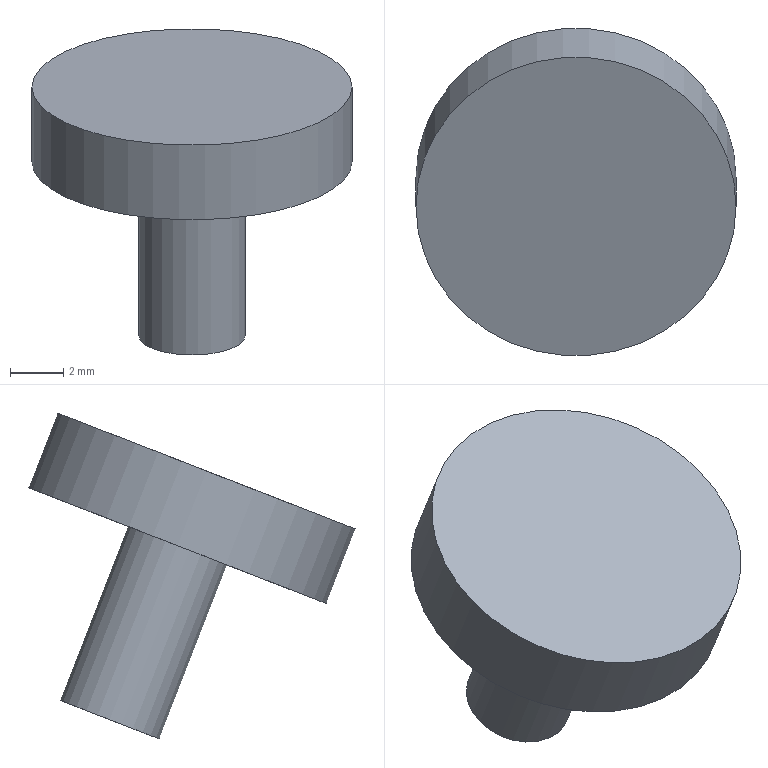Component | NX | 23G__27 | 1 solid | 5 faces | box 12 x 12.27 x 12.22 mm | volume 427 mm3 | plane 3 | cylinder 2 | commonest cylinder face diameters 4 x1 12 x1
STEP:
#1=CARTESIAN_POINT('',(0.,0.,0.));
#2=DIRECTION('',(0.,0.,1.));
#3=DIRECTION('',(1.,0.,0.));
#4=AXIS2_PLACEMENT_3D('',#1,#2,#3);
#5=CARTESIAN_POINT('',(19.022,57.969,101.64));
#6=VERTEX_POINT('',#5);
#7=CARTESIAN_POINT('',(17.022,57.969,101.64));
#8=DIRECTION('',(0.,-0.3629,0.9318));
#9=DIRECTION('',(1.,0.,0.));
#10=AXIS2_PLACEMENT_3D('',#7,#8,#9);
#11=CIRCLE('',#10,2.);
#12=CARTESIAN_POINT('',(17.022,57.969,101.64));
#13=DIRECTION('',(0.,-0.3629,0.9318));
#14=DIRECTION('',(1.,0.,0.));
#15=AXIS2_PLACEMENT_3D('',#12,#13,#14);
#16=PLANE('',#15);
#17=CARTESIAN_POINT('',(0.,0.));
#18=DIRECTION('',(1.,0.));
#19=AXIS2_PLACEMENT_2D('',#17,#18);
#20=CIRCLE('',#19,2.);
#21=(GEOMETRIC_REPRESENTATION_CONTEXT(2)PARAMETRIC_REPRESENTATION_CONTEXT()REPRESENTATION_CONTEXT('',''));
#22=DEFINITIONAL_REPRESENTATION('',(#20),#21);
#23=PCURVE('',#16,#22);
#24=CARTESIAN_POINT('',(17.022,57.969,101.64));
#25=DIRECTION('',(0.,-0.3629,0.9318));
#26=DIRECTION('',(1.,0.,0.));
#27=AXIS2_PLACEMENT_3D('',#24,#25,#26);
#28=CYLINDRICAL_SURFACE('',#27,2.);
#29=CARTESIAN_POINT('',(0.,0.));
#30=DIRECTION('',(1.,0.));
#31=VECTOR('',#30,1.);
#32=LINE('',#29,#31);
#33=(GEOMETRIC_REPRESENTATION_CONTEXT(2)PARAMETRIC_REPRESENTATION_CONTEXT()REPRESENTATION_CONTEXT('',''));
#34=DEFINITIONAL_REPRESENTATION('',(#32),#33);
#35=PCURVE('',#28,#34);
#36=SURFACE_CURVE('',#11,(#23,#35),.PCURVE_S1.);
#37=EDGE_CURVE('',#6,#6,#36,.T.);
#38=ORIENTED_EDGE('',*,*,#37,.F.);
#39=EDGE_LOOP('',(#38));
#40=FACE_BOUND('',#39,.T.);
#41=ADVANCED_FACE('',(#40),#16,.F.);
#42=CARTESIAN_POINT('',(19.022,55.429,108.162));
#43=VERTEX_POINT('',#42);
#44=CARTESIAN_POINT('',(17.022,55.429,108.162));
#45=DIRECTION('',(0.,-0.3629,0.9318));
#46=DIRECTION('',(1.,0.,0.));
#47=AXIS2_PLACEMENT_3D('',#44,#45,#46);
#48=CIRCLE('',#47,2.);
#49=CARTESIAN_POINT('',(0.,7.));
#50=DIRECTION('',(1.,0.));
#51=VECTOR('',#50,1.);
#52=LINE('',#49,#51);
#53=(GEOMETRIC_REPRESENTATION_CONTEXT(2)PARAMETRIC_REPRESENTATION_CONTEXT()REPRESENTATION_CONTEXT('',''));
#54=DEFINITIONAL_REPRESENTATION('',(#52),#53);
#55=PCURVE('',#28,#54);
#56=CARTESIAN_POINT('',(17.022,57.292,108.888));
#57=DIRECTION('',(0.,-0.3629,0.9318));
#58=DIRECTION('',(1.,0.,0.));
#59=AXIS2_PLACEMENT_3D('',#56,#57,#58);
#60=PLANE('',#59);
#61=CARTESIAN_POINT('',(0.,-2.));
#62=DIRECTION('',(1.,0.));
#63=AXIS2_PLACEMENT_2D('',#61,#62);
#64=CIRCLE('',#63,2.);
#65=(GEOMETRIC_REPRESENTATION_CONTEXT(2)PARAMETRIC_REPRESENTATION_CONTEXT()REPRESENTATION_CONTEXT('',''));
#66=DEFINITIONAL_REPRESENTATION('',(#64),#65);
#67=PCURVE('',#60,#66);
#68=SURFACE_CURVE('',#48,(#55,#67),.PCURVE_S1.);
#69=EDGE_CURVE('',#43,#43,#68,.T.);
#70=ORIENTED_EDGE('',*,*,#69,.F.);
#71=CARTESIAN_POINT('',(19.022,57.969,101.64));
#72=CARTESIAN_POINT('',(19.022,55.429,108.162));
#73=B_SPLINE_CURVE_WITH_KNOTS('',1,(#71,#72),.UNSPECIFIED.,.F.,.F.,(2,2),(0.,7.),.PIECEWISE_BEZIER_KNOTS.);
#74=CARTESIAN_POINT('',(0.,0.));
#75=DIRECTION('',(0.,1.));
#76=VECTOR('',#75,1.);
#77=LINE('',#74,#76);
#78=(GEOMETRIC_REPRESENTATION_CONTEXT(2)PARAMETRIC_REPRESENTATION_CONTEXT()REPRESENTATION_CONTEXT('',''));
#79=DEFINITIONAL_REPRESENTATION('',(#77),#78);
#80=PCURVE('',#28,#79);
#81=CARTESIAN_POINT('',(6.283,0.));
#82=DIRECTION('',(0.,1.));
#83=VECTOR('',#82,1.);
#84=LINE('',#81,#83);
#85=(GEOMETRIC_REPRESENTATION_CONTEXT(2)PARAMETRIC_REPRESENTATION_CONTEXT()REPRESENTATION_CONTEXT('',''));
#86=DEFINITIONAL_REPRESENTATION('',(#84),#85);
#87=PCURVE('',#28,#86);
#88=SEAM_CURVE('',#73,(#80,#87),.PCURVE_S1.);
#89=EDGE_CURVE('',#6,#43,#88,.T.);
#90=ORIENTED_EDGE('',*,*,#89,.F.);
#91=ORIENTED_EDGE('',*,*,#37,.T.);
#92=ORIENTED_EDGE('',*,*,#89,.T.);
#93=EDGE_LOOP('',(#70,#90,#91,#92));
#94=FACE_BOUND('',#93,.T.);
#95=ADVANCED_FACE('',(#94),#28,.T.);
#96=CARTESIAN_POINT('',(23.022,55.429,108.162));
#97=VERTEX_POINT('',#96);
#98=CARTESIAN_POINT('',(17.022,55.429,108.162));
#99=DIRECTION('',(0.,-0.3629,0.9318));
#100=DIRECTION('',(1.,0.,0.));
#101=AXIS2_PLACEMENT_3D('',#98,#99,#100);
#102=CIRCLE('',#101,6.);
#103=CARTESIAN_POINT('',(0.,-2.));
#104=DIRECTION('',(1.,0.));
#105=AXIS2_PLACEMENT_2D('',#103,#104);
#106=CIRCLE('',#105,6.);
#107=(GEOMETRIC_REPRESENTATION_CONTEXT(2)PARAMETRIC_REPRESENTATION_CONTEXT()REPRESENTATION_CONTEXT('',''));
#108=DEFINITIONAL_REPRESENTATION('',(#106),#107);
#109=PCURVE('',#60,#108);
#110=CARTESIAN_POINT('',(17.022,57.969,101.64));
#111=DIRECTION('',(0.,-0.3629,0.9318));
#112=DIRECTION('',(1.,0.,0.));
#113=AXIS2_PLACEMENT_3D('',#110,#111,#112);
#114=CYLINDRICAL_SURFACE('',#113,6.);
#115=CARTESIAN_POINT('',(0.,7.));
#116=DIRECTION('',(1.,0.));
#117=VECTOR('',#116,1.);
#118=LINE('',#115,#117);
#119=(GEOMETRIC_REPRESENTATION_CONTEXT(2)PARAMETRIC_REPRESENTATION_CONTEXT()REPRESENTATION_CONTEXT('',''));
#120=DEFINITIONAL_REPRESENTATION('',(#118),#119);
#121=PCURVE('',#114,#120);
#122=SURFACE_CURVE('',#102,(#109,#121),.PCURVE_S1.);
#123=EDGE_CURVE('',#97,#97,#122,.T.);
#124=ORIENTED_EDGE('',*,*,#123,.F.);
#125=EDGE_LOOP('',(#124));
#126=FACE_BOUND('',#125,.T.);
#127=ORIENTED_EDGE('',*,*,#69,.T.);
#128=EDGE_LOOP('',(#127));
#129=FACE_BOUND('',#128,.T.);
#130=ADVANCED_FACE('',(#126,#129),#60,.F.);
#131=CARTESIAN_POINT('',(23.022,54.34,110.958));
#132=VERTEX_POINT('',#131);
#133=CARTESIAN_POINT('',(17.022,54.34,110.958));
#134=DIRECTION('',(0.,-0.3629,0.9318));
#135=DIRECTION('',(1.,0.,0.));
#136=AXIS2_PLACEMENT_3D('',#133,#134,#135);
#137=CIRCLE('',#136,6.);
#138=CARTESIAN_POINT('',(0.,10.));
#139=DIRECTION('',(1.,0.));
#140=VECTOR('',#139,1.);
#141=LINE('',#138,#140);
#142=(GEOMETRIC_REPRESENTATION_CONTEXT(2)PARAMETRIC_REPRESENTATION_CONTEXT()REPRESENTATION_CONTEXT('',''));
#143=DEFINITIONAL_REPRESENTATION('',(#141),#142);
#144=PCURVE('',#114,#143);
#145=CARTESIAN_POINT('',(17.022,59.931,113.135));
#146=DIRECTION('',(0.,0.3629,-0.9318));
#147=DIRECTION('',(-1.,0.,0.));
#148=AXIS2_PLACEMENT_3D('',#145,#146,#147);
#149=PLANE('',#148);
#150=CARTESIAN_POINT('',(-6.,-6.));
#151=CARTESIAN_POINT('',(-6.,4.392));
#152=CARTESIAN_POINT('',(3.,-0.8038));
#153=CARTESIAN_POINT('',(12.,-6.));
#154=CARTESIAN_POINT('',(3.,-11.196));
#155=CARTESIAN_POINT('',(-6.,-16.392));
#156=CARTESIAN_POINT('',(-6.,-6.));
#157=(BOUNDED_CURVE()B_SPLINE_CURVE(2,(#150,#151,#152,#153,#154,#155,#156),.UNSPECIFIED.,.T.,.F.)B_SPLINE_CURVE_WITH_KNOTS((1,2,2,2,2,1),(-2.094,0.,2.094,4.189,6.283,8.378),.UNSPECIFIED.)CURVE()GEOMETRIC_REPRESENTATION_ITEM()RATIONAL_B_SPLINE_CURVE((1.,0.5,1.,0.5,1.,0.5,1.))REPRESENTATION_ITEM(''));
#158=(GEOMETRIC_REPRESENTATION_CONTEXT(2)PARAMETRIC_REPRESENTATION_CONTEXT()REPRESENTATION_CONTEXT('',''));
#159=DEFINITIONAL_REPRESENTATION('',(#157),#158);
#160=PCURVE('',#149,#159);
#161=SURFACE_CURVE('',#137,(#144,#160),.PCURVE_S1.);
#162=EDGE_CURVE('',#132,#132,#161,.T.);
#163=ORIENTED_EDGE('',*,*,#162,.F.);
#164=CARTESIAN_POINT('',(23.022,55.429,108.162));
#165=CARTESIAN_POINT('',(23.022,54.34,110.958));
#166=B_SPLINE_CURVE_WITH_KNOTS('',1,(#164,#165),.UNSPECIFIED.,.F.,.F.,(2,2),(7.,10.),.PIECEWISE_BEZIER_KNOTS.);
#167=CARTESIAN_POINT('',(0.,0.));
#168=DIRECTION('',(0.,1.));
#169=VECTOR('',#168,1.);
#170=LINE('',#167,#169);
#171=(GEOMETRIC_REPRESENTATION_CONTEXT(2)PARAMETRIC_REPRESENTATION_CONTEXT()REPRESENTATION_CONTEXT('',''));
#172=DEFINITIONAL_REPRESENTATION('',(#170),#171);
#173=PCURVE('',#114,#172);
#174=CARTESIAN_POINT('',(6.283,0.));
#175=DIRECTION('',(0.,1.));
#176=VECTOR('',#175,1.);
#177=LINE('',#174,#176);
#178=(GEOMETRIC_REPRESENTATION_CONTEXT(2)PARAMETRIC_REPRESENTATION_CONTEXT()REPRESENTATION_CONTEXT('',''));
#179=DEFINITIONAL_REPRESENTATION('',(#177),#178);
#180=PCURVE('',#114,#179);
#181=SEAM_CURVE('',#166,(#173,#180),.PCURVE_S1.);
#182=EDGE_CURVE('',#97,#132,#181,.T.);
#183=ORIENTED_EDGE('',*,*,#182,.F.);
#184=ORIENTED_EDGE('',*,*,#123,.T.);
#185=ORIENTED_EDGE('',*,*,#182,.T.);
#186=EDGE_LOOP('',(#163,#183,#184,#185));
#187=FACE_BOUND('',#186,.T.);
#188=ADVANCED_FACE('',(#187),#114,.T.);
#189=ORIENTED_EDGE('',*,*,#162,.T.);
#190=EDGE_LOOP('',(#189));
#191=FACE_BOUND('',#190,.T.);
#192=ADVANCED_FACE('',(#191),#149,.F.);
#193=CLOSED_SHELL('',(#41,#95,#130,#188,#192));
#194=MANIFOLD_SOLID_BREP('',#193);
#195=(LENGTH_UNIT()NAMED_UNIT(*)SI_UNIT(.MILLI.,.METRE.));
#196=UNCERTAINTY_MEASURE_WITH_UNIT(LENGTH_MEASURE(0.00001),#195,'','');
#197=(NAMED_UNIT(*)PLANE_ANGLE_UNIT()SI_UNIT($,.RADIAN.));
#198=(NAMED_UNIT(*)SI_UNIT($,.STERADIAN.)SOLID_ANGLE_UNIT());
#199=(GEOMETRIC_REPRESENTATION_CONTEXT(3)GLOBAL_UNCERTAINTY_ASSIGNED_CONTEXT((#196))GLOBAL_UNIT_ASSIGNED_CONTEXT((#195,#197,#198))REPRESENTATION_CONTEXT('',''));
#200=ADVANCED_BREP_SHAPE_REPRESENTATION('',(#4,#194),#199);